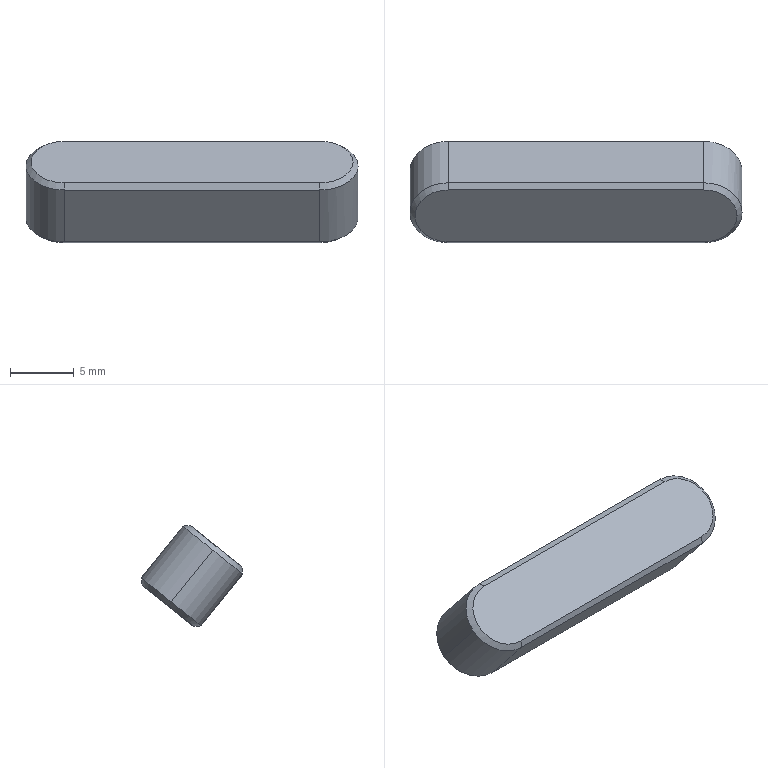Component | SolidWorks | Key6-6-32-1 | 1 solid | 17 faces | box 26 x 7.93 x 7.93 mm | volume 880 mm3 | plane 8 | cone 6 | cylinder 3 | commonest cylinder face diameters 6 x3
build123d program:
from build123d import *

# Parameters (mm, degrees)
BOSS_EXTRUDE1_DEPTH = 6
CHAMFER1_SIZE2      = 0.4
CHAMFER1_SIZE       = 0.4


with BuildPart() as part:
    # Sketch1 → Boss-Extrude1 (new body)
    with BuildSketch(Plane(origin=(0, 0, 4), x_dir=(1, 0, 0), z_dir=(0, -1, 0))):
        with BuildLine():
            Line((-3, 16), (-3, -4))
            ThreePointArc((-3, -4), (0, -7), (3, -4))
            Line((3, -4), (3, 16))
            ThreePointArc((3, 16), (0, 19), (-3, 16))
        make_face()
    extrude(amount=-BOSS_EXTRUDE1_DEPTH)

    # Chamfer1
    chamfer1_edges = [part.edges().sort_by_distance(p)[0] for p in [
        (0, 6, -3),
        (3, 6, 10),
        (0, 6, 23),
        (3, 0, 10),
        (0, 0, -3),
        (-3, 0, 10),
        (0, 0, 23),
        (-3, 6, 10),
    ]]
    chamfer(chamfer1_edges, length=CHAMFER1_SIZE, length2=CHAMFER1_SIZE2)


solid = part.part

# Placed as in the assembly
solid = solid.moved(Location((-300.42, 4.252, -5.306), (-51.293, -90, 0)))
STEP:
#1=COLOUR_RGB('',0.7922,0.8196,0.9333);
#2=FILL_AREA_STYLE_COLOUR('',#1);
#3=FILL_AREA_STYLE('',(#2));
#4=SURFACE_STYLE_FILL_AREA(#3);
#5=SURFACE_SIDE_STYLE('',(#4));
#6=SURFACE_STYLE_USAGE(.BOTH.,#5);
#7=PRESENTATION_STYLE_ASSIGNMENT((#6));
#8=CARTESIAN_POINT('',(-12.717,0.3151,-0.3932));
#9=VERTEX_POINT('',#8);
#10=CARTESIAN_POINT('',(-12.615,0.395,-0.3292));
#11=VERTEX_POINT('',#10);
#12=CARTESIAN_POINT('',(-12.615,0.3151,-0.3932));
#13=DIRECTION('',(-0.,0.6253,-0.7803));
#14=DIRECTION('',(-1.,0.,0.));
#15=AXIS2_PLACEMENT_3D('',#12,#13,#14);
#16=CIRCLE('',#15,0.1024);
#17=EDGE_CURVE('',#9,#11,#16,.T.);
#18=ORIENTED_EDGE('',*,*,#17,.F.);
#19=CARTESIAN_POINT('',(-12.733,0.3053,-0.381));
#20=VERTEX_POINT('',#19);
#21=CARTESIAN_POINT('',(-12.733,0.3053,-0.381));
#22=DIRECTION('',(-0.7071,-0.4422,0.5518));
#23=VECTOR('',#22,39.37);
#24=LINE('',#21,#23);
#25=EDGE_CURVE('',#9,#20,#24,.T.);
#26=ORIENTED_EDGE('',*,*,#25,.T.);
#27=CARTESIAN_POINT('',(-12.615,0.3975,-0.3071));
#28=VERTEX_POINT('',#27);
#29=CARTESIAN_POINT('',(-12.615,0.3053,-0.381));
#30=DIRECTION('',(0.,-0.6253,0.7803));
#31=DIRECTION('',(-1.,-0.,0.));
#32=AXIS2_PLACEMENT_3D('',#29,#30,#31);
#33=CIRCLE('',#32,0.1181);
#34=EDGE_CURVE('',#28,#20,#33,.T.);
#35=ORIENTED_EDGE('',*,*,#34,.F.);
#36=CARTESIAN_POINT('',(-12.615,0.395,-0.3292));
#37=DIRECTION('',(0.,0.1096,0.994));
#38=VECTOR('',#37,39.37);
#39=LINE('',#36,#38);
#40=EDGE_CURVE('',#11,#28,#39,.T.);
#41=ORIENTED_EDGE('',*,*,#40,.F.);
#42=EDGE_LOOP('',(#18,#26,#35,#41));
#43=FACE_OUTER_BOUND('',#42,.T.);
#44=CARTESIAN_POINT('',(-12.615,0.3053,-0.381));
#45=DIRECTION('',(0.,-0.6253,0.7803));
#46=DIRECTION('',(-1.,-0.,0.));
#47=AXIS2_PLACEMENT_3D('',#44,#45,#46);
#48=CONICAL_SURFACE('',#47,0.1181,0.7854);
#49=ADVANCED_FACE('',(#43),#48,.T.);
#50=CARTESIAN_POINT('',(-11.725,0.1674,-0.2089));
#51=VERTEX_POINT('',#50);
#52=CARTESIAN_POINT('',(-11.828,0.2473,-0.1449));
#53=VERTEX_POINT('',#52);
#54=CARTESIAN_POINT('',(-11.828,0.1674,-0.2089));
#55=DIRECTION('',(0.,-0.6253,0.7803));
#56=DIRECTION('',(-1.,-0.,0.));
#57=AXIS2_PLACEMENT_3D('',#54,#55,#56);
#58=CIRCLE('',#57,0.1024);
#59=EDGE_CURVE('',#51,#53,#58,.T.);
#60=ORIENTED_EDGE('',*,*,#59,.F.);
#61=CARTESIAN_POINT('',(-11.709,0.1773,-0.2212));
#62=VERTEX_POINT('',#61);
#63=CARTESIAN_POINT('',(-11.725,0.1674,-0.2089));
#64=DIRECTION('',(0.7071,0.4422,-0.5518));
#65=VECTOR('',#64,39.37);
#66=LINE('',#63,#65);
#67=EDGE_CURVE('',#51,#62,#66,.T.);
#68=ORIENTED_EDGE('',*,*,#67,.T.);
#69=CARTESIAN_POINT('',(-11.828,0.2694,-0.1473));
#70=VERTEX_POINT('',#69);
#71=CARTESIAN_POINT('',(-11.828,0.1773,-0.2212));
#72=DIRECTION('',(-0.,0.6253,-0.7803));
#73=DIRECTION('',(-1.,-0.,0.));
#74=AXIS2_PLACEMENT_3D('',#71,#72,#73);
#75=CIRCLE('',#74,0.1181);
#76=EDGE_CURVE('',#70,#62,#75,.T.);
#77=ORIENTED_EDGE('',*,*,#76,.F.);
#78=CARTESIAN_POINT('',(-11.828,0.2694,-0.1473));
#79=DIRECTION('',(0.,-0.994,0.1096));
#80=VECTOR('',#79,39.37);
#81=LINE('',#78,#80);
#82=EDGE_CURVE('',#70,#53,#81,.T.);
#83=ORIENTED_EDGE('',*,*,#82,.T.);
#84=EDGE_LOOP('',(#60,#68,#77,#83));
#85=FACE_OUTER_BOUND('',#84,.T.);
#86=CARTESIAN_POINT('',(-11.828,0.1674,-0.2089));
#87=DIRECTION('',(-0.,0.6253,-0.7803));
#88=DIRECTION('',(1.,0.,0.));
#89=AXIS2_PLACEMENT_3D('',#86,#87,#88);
#90=CONICAL_SURFACE('',#89,0.1024,0.7854);
#91=ADVANCED_FACE('',(#85),#90,.T.);
#92=ORIENTED_EDGE('',*,*,#34,.T.);
#93=CARTESIAN_POINT('',(-12.733,0.1773,-0.2212));
#94=VERTEX_POINT('',#93);
#95=CARTESIAN_POINT('',(-12.733,0.3151,-0.3932));
#96=DIRECTION('',(0.,-0.6253,0.7803));
#97=VECTOR('',#96,39.37);
#98=LINE('',#95,#97);
#99=EDGE_CURVE('',#20,#94,#98,.T.);
#100=ORIENTED_EDGE('',*,*,#99,.T.);
#101=CARTESIAN_POINT('',(-12.615,0.2694,-0.1473));
#102=VERTEX_POINT('',#101);
#103=CARTESIAN_POINT('',(-12.615,0.1773,-0.2212));
#104=DIRECTION('',(-0.,0.6253,-0.7803));
#105=DIRECTION('',(-1.,-0.,0.));
#106=AXIS2_PLACEMENT_3D('',#103,#104,#105);
#107=CIRCLE('',#106,0.1181);
#108=EDGE_CURVE('',#94,#102,#107,.T.);
#109=ORIENTED_EDGE('',*,*,#108,.T.);
#110=CARTESIAN_POINT('',(-12.615,0.4073,-0.3194));
#111=DIRECTION('',(0.,-0.6253,0.7803));
#112=VECTOR('',#111,39.37);
#113=LINE('',#110,#112);
#114=EDGE_CURVE('',#28,#102,#113,.T.);
#115=ORIENTED_EDGE('',*,*,#114,.F.);
#116=EDGE_LOOP('',(#92,#100,#109,#115));
#117=FACE_OUTER_BOUND('',#116,.T.);
#118=CARTESIAN_POINT('',(-12.615,0.3151,-0.3932));
#119=DIRECTION('',(0.,-0.6253,0.7803));
#120=DIRECTION('',(-1.,0.,0.));
#121=AXIS2_PLACEMENT_3D('',#118,#119,#120);
#122=CYLINDRICAL_SURFACE('',#121,0.1181);
#123=ADVANCED_FACE('',(#117),#122,.T.);
#124=CARTESIAN_POINT('',(-11.828,0.3975,-0.3071));
#125=VERTEX_POINT('',#124);
#126=CARTESIAN_POINT('',(-11.828,0.4073,-0.3194));
#127=DIRECTION('',(0.,-0.6253,0.7803));
#128=VECTOR('',#127,39.37);
#129=LINE('',#126,#128);
#130=EDGE_CURVE('',#125,#70,#129,.T.);
#131=ORIENTED_EDGE('',*,*,#130,.T.);
#132=ORIENTED_EDGE('',*,*,#76,.T.);
#133=CARTESIAN_POINT('',(-11.828,0.0851,-0.2951));
#134=VERTEX_POINT('',#133);
#135=CARTESIAN_POINT('',(-11.828,0.1773,-0.2212));
#136=DIRECTION('',(-0.,0.6253,-0.7803));
#137=DIRECTION('',(-1.,-0.,0.));
#138=AXIS2_PLACEMENT_3D('',#135,#136,#137);
#139=CIRCLE('',#138,0.1181);
#140=EDGE_CURVE('',#62,#134,#139,.T.);
#141=ORIENTED_EDGE('',*,*,#140,.T.);
#142=CARTESIAN_POINT('',(-11.828,0.2131,-0.4548));
#143=VERTEX_POINT('',#142);
#144=CARTESIAN_POINT('',(-11.828,0.223,-0.4671));
#145=DIRECTION('',(0.,-0.6253,0.7803));
#146=VECTOR('',#145,39.37);
#147=LINE('',#144,#146);
#148=EDGE_CURVE('',#143,#134,#147,.T.);
#149=ORIENTED_EDGE('',*,*,#148,.F.);
#150=CARTESIAN_POINT('',(-11.828,0.3053,-0.381));
#151=DIRECTION('',(0.,-0.6253,0.7803));
#152=DIRECTION('',(-1.,-0.,0.));
#153=AXIS2_PLACEMENT_3D('',#150,#151,#152);
#154=CIRCLE('',#153,0.1181);
#155=EDGE_CURVE('',#143,#125,#154,.T.);
#156=ORIENTED_EDGE('',*,*,#155,.T.);
#157=EDGE_LOOP('',(#131,#132,#141,#149,#156));
#158=FACE_OUTER_BOUND('',#157,.T.);
#159=CARTESIAN_POINT('',(-11.828,0.3151,-0.3932));
#160=DIRECTION('',(0.,-0.6253,0.7803));
#161=DIRECTION('',(-1.,0.,0.));
#162=AXIS2_PLACEMENT_3D('',#159,#160,#161);
#163=CYLINDRICAL_SURFACE('',#162,0.1181);
#164=ADVANCED_FACE('',(#158),#163,.T.);
#165=ORIENTED_EDGE('',*,*,#148,.T.);
#166=CARTESIAN_POINT('',(-12.615,0.0851,-0.2951));
#167=VERTEX_POINT('',#166);
#168=CARTESIAN_POINT('',(-12.615,0.0851,-0.2951));
#169=DIRECTION('',(-1.,0.,0.));
#170=VECTOR('',#169,39.37);
#171=LINE('',#168,#170);
#172=EDGE_CURVE('',#134,#167,#171,.T.);
#173=ORIENTED_EDGE('',*,*,#172,.T.);
#174=CARTESIAN_POINT('',(-12.615,0.2131,-0.4548));
#175=VERTEX_POINT('',#174);
#176=CARTESIAN_POINT('',(-12.615,0.223,-0.4671));
#177=DIRECTION('',(0.,-0.6253,0.7803));
#178=VECTOR('',#177,39.37);
#179=LINE('',#176,#178);
#180=EDGE_CURVE('',#175,#167,#179,.T.);
#181=ORIENTED_EDGE('',*,*,#180,.F.);
#182=CARTESIAN_POINT('',(-11.828,0.2131,-0.4548));
#183=DIRECTION('',(1.,-0.,-0.));
#184=VECTOR('',#183,39.37);
#185=LINE('',#182,#184);
#186=EDGE_CURVE('',#175,#143,#185,.T.);
#187=ORIENTED_EDGE('',*,*,#186,.T.);
#188=EDGE_LOOP('',(#165,#173,#181,#187));
#189=FACE_OUTER_BOUND('',#188,.T.);
#190=CARTESIAN_POINT('',(-12.615,0.223,-0.4671));
#191=DIRECTION('',(-0.,-0.7803,-0.6253));
#192=DIRECTION('',(-1.,0.,0.));
#193=AXIS2_PLACEMENT_3D('',#190,#191,#192);
#194=PLANE('',#193);
#195=ADVANCED_FACE('',(#189),#194,.T.);
#196=ORIENTED_EDGE('',*,*,#99,.F.);
#197=CARTESIAN_POINT('',(-12.615,0.3053,-0.381));
#198=DIRECTION('',(0.,-0.6253,0.7803));
#199=DIRECTION('',(-1.,-0.,0.));
#200=AXIS2_PLACEMENT_3D('',#197,#198,#199);
#201=CIRCLE('',#200,0.1181);
#202=EDGE_CURVE('',#20,#175,#201,.T.);
#203=ORIENTED_EDGE('',*,*,#202,.T.);
#204=ORIENTED_EDGE('',*,*,#180,.T.);
#205=CARTESIAN_POINT('',(-12.615,0.1773,-0.2212));
#206=DIRECTION('',(-0.,0.6253,-0.7803));
#207=DIRECTION('',(-1.,0.,0.));
#208=AXIS2_PLACEMENT_3D('',#205,#206,#207);
#209=CIRCLE('',#208,0.1181);
#210=EDGE_CURVE('',#167,#94,#209,.T.);
#211=ORIENTED_EDGE('',*,*,#210,.T.);
#212=EDGE_LOOP('',(#196,#203,#204,#211));
#213=FACE_OUTER_BOUND('',#212,.T.);
#214=CARTESIAN_POINT('',(-12.615,0.3151,-0.3932));
#215=DIRECTION('',(0.,-0.6253,0.7803));
#216=DIRECTION('',(-1.,0.,0.));
#217=AXIS2_PLACEMENT_3D('',#214,#215,#216);
#218=CYLINDRICAL_SURFACE('',#217,0.1181);
#219=ADVANCED_FACE('',(#213),#218,.T.);
#220=ORIENTED_EDGE('',*,*,#114,.T.);
#221=CARTESIAN_POINT('',(-11.828,0.2694,-0.1473));
#222=DIRECTION('',(1.,-0.,-0.));
#223=VECTOR('',#222,39.37);
#224=LINE('',#221,#223);
#225=EDGE_CURVE('',#102,#70,#224,.T.);
#226=ORIENTED_EDGE('',*,*,#225,.T.);
#227=ORIENTED_EDGE('',*,*,#130,.F.);
#228=CARTESIAN_POINT('',(-12.615,0.3975,-0.3071));
#229=DIRECTION('',(-1.,0.,0.));
#230=VECTOR('',#229,39.37);
#231=LINE('',#228,#230);
#232=EDGE_CURVE('',#125,#28,#231,.T.);
#233=ORIENTED_EDGE('',*,*,#232,.T.);
#234=EDGE_LOOP('',(#220,#226,#227,#233));
#235=FACE_OUTER_BOUND('',#234,.T.);
#236=CARTESIAN_POINT('',(-11.828,0.4073,-0.3194));
#237=DIRECTION('',(0.,0.7803,0.6253));
#238=DIRECTION('',(1.,-0.,-0.));
#239=AXIS2_PLACEMENT_3D('',#236,#237,#238);
#240=PLANE('',#239);
#241=ADVANCED_FACE('',(#235),#240,.T.);
#242=CARTESIAN_POINT('',(-12.615,0.2353,-0.4573));
#243=VERTEX_POINT('',#242);
#244=CARTESIAN_POINT('',(-12.615,0.3151,-0.3932));
#245=DIRECTION('',(-0.,0.6253,-0.7803));
#246=DIRECTION('',(-1.,0.,0.));
#247=AXIS2_PLACEMENT_3D('',#244,#245,#246);
#248=CIRCLE('',#247,0.1024);
#249=EDGE_CURVE('',#243,#9,#248,.T.);
#250=ORIENTED_EDGE('',*,*,#249,.T.);
#251=ORIENTED_EDGE('',*,*,#17,.T.);
#252=CARTESIAN_POINT('',(-11.828,0.395,-0.3292));
#253=VERTEX_POINT('',#252);
#254=CARTESIAN_POINT('',(-11.828,0.395,-0.3292));
#255=DIRECTION('',(1.,-0.,-0.));
#256=VECTOR('',#255,39.37);
#257=LINE('',#254,#256);
#258=EDGE_CURVE('',#11,#253,#257,.T.);
#259=ORIENTED_EDGE('',*,*,#258,.T.);
#260=CARTESIAN_POINT('',(-11.828,0.2353,-0.4573));
#261=VERTEX_POINT('',#260);
#262=CARTESIAN_POINT('',(-11.828,0.3151,-0.3932));
#263=DIRECTION('',(-0.,0.6253,-0.7803));
#264=DIRECTION('',(-1.,0.,0.));
#265=AXIS2_PLACEMENT_3D('',#262,#263,#264);
#266=CIRCLE('',#265,0.1024);
#267=EDGE_CURVE('',#253,#261,#266,.T.);
#268=ORIENTED_EDGE('',*,*,#267,.T.);
#269=CARTESIAN_POINT('',(-12.615,0.2353,-0.4573));
#270=DIRECTION('',(-1.,0.,0.));
#271=VECTOR('',#270,39.37);
#272=LINE('',#269,#271);
#273=EDGE_CURVE('',#261,#243,#272,.T.);
#274=ORIENTED_EDGE('',*,*,#273,.T.);
#275=EDGE_LOOP('',(#250,#251,#259,#268,#274));
#276=FACE_OUTER_BOUND('',#275,.T.);
#277=CARTESIAN_POINT('',(-11.828,0.3151,-0.3932));
#278=DIRECTION('',(-0.,-0.6253,0.7803));
#279=DIRECTION('',(-1.,-0.,-0.));
#280=AXIS2_PLACEMENT_3D('',#277,#278,#279);
#281=PLANE('',#280);
#282=ADVANCED_FACE('',(#276),#281,.F.);
#283=CARTESIAN_POINT('',(-12.615,0.2473,-0.1449));
#284=VERTEX_POINT('',#283);
#285=CARTESIAN_POINT('',(-12.615,0.08754,-0.2729));
#286=VERTEX_POINT('',#285);
#287=CARTESIAN_POINT('',(-12.615,0.1674,-0.2089));
#288=DIRECTION('',(0.,-0.6253,0.7803));
#289=DIRECTION('',(-1.,-0.,0.));
#290=AXIS2_PLACEMENT_3D('',#287,#288,#289);
#291=CIRCLE('',#290,0.1024);
#292=EDGE_CURVE('',#284,#286,#291,.T.);
#293=ORIENTED_EDGE('',*,*,#292,.T.);
#294=CARTESIAN_POINT('',(-11.828,0.08754,-0.2729));
#295=VERTEX_POINT('',#294);
#296=CARTESIAN_POINT('',(-11.828,0.08754,-0.2729));
#297=DIRECTION('',(1.,-0.,-0.));
#298=VECTOR('',#297,39.37);
#299=LINE('',#296,#298);
#300=EDGE_CURVE('',#286,#295,#299,.T.);
#301=ORIENTED_EDGE('',*,*,#300,.T.);
#302=CARTESIAN_POINT('',(-11.828,0.1674,-0.2089));
#303=DIRECTION('',(0.,-0.6253,0.7803));
#304=DIRECTION('',(-1.,-0.,0.));
#305=AXIS2_PLACEMENT_3D('',#302,#303,#304);
#306=CIRCLE('',#305,0.1024);
#307=EDGE_CURVE('',#295,#51,#306,.T.);
#308=ORIENTED_EDGE('',*,*,#307,.T.);
#309=ORIENTED_EDGE('',*,*,#59,.T.);
#310=CARTESIAN_POINT('',(-11.828,0.2473,-0.1449));
#311=DIRECTION('',(-1.,0.,0.));
#312=VECTOR('',#311,39.37);
#313=LINE('',#310,#312);
#314=EDGE_CURVE('',#53,#284,#313,.T.);
#315=ORIENTED_EDGE('',*,*,#314,.T.);
#316=EDGE_LOOP('',(#293,#301,#308,#309,#315));
#317=FACE_OUTER_BOUND('',#316,.T.);
#318=CARTESIAN_POINT('',(-11.828,0.1674,-0.2089));
#319=DIRECTION('',(-0.,-0.6253,0.7803));
#320=DIRECTION('',(-1.,-0.,-0.));
#321=AXIS2_PLACEMENT_3D('',#318,#319,#320);
#322=PLANE('',#321);
#323=ADVANCED_FACE('',(#317),#322,.T.);
#324=ORIENTED_EDGE('',*,*,#82,.F.);
#325=ORIENTED_EDGE('',*,*,#225,.F.);
#326=CARTESIAN_POINT('',(-12.615,0.2473,-0.1449));
#327=DIRECTION('',(-0.,0.994,-0.1096));
#328=VECTOR('',#327,39.37);
#329=LINE('',#326,#328);
#330=EDGE_CURVE('',#284,#102,#329,.T.);
#331=ORIENTED_EDGE('',*,*,#330,.F.);
#332=ORIENTED_EDGE('',*,*,#314,.F.);
#333=EDGE_LOOP('',(#324,#325,#331,#332));
#334=FACE_OUTER_BOUND('',#333,.T.);
#335=CARTESIAN_POINT('',(-11.828,0.2473,-0.1449));
#336=DIRECTION('',(-0.,-0.1096,-0.994));
#337=DIRECTION('',(-1.,0.,0.));
#338=AXIS2_PLACEMENT_3D('',#335,#336,#337);
#339=PLANE('',#338);
#340=ADVANCED_FACE('',(#334),#339,.F.);
#341=ORIENTED_EDGE('',*,*,#330,.T.);
#342=ORIENTED_EDGE('',*,*,#108,.F.);
#343=ORIENTED_EDGE('',*,*,#210,.F.);
#344=CARTESIAN_POINT('',(-12.615,0.08754,-0.2729));
#345=DIRECTION('',(-0.,-0.1096,-0.994));
#346=VECTOR('',#345,39.37);
#347=LINE('',#344,#346);
#348=EDGE_CURVE('',#286,#167,#347,.T.);
#349=ORIENTED_EDGE('',*,*,#348,.F.);
#350=ORIENTED_EDGE('',*,*,#292,.F.);
#351=EDGE_LOOP('',(#341,#342,#343,#349,#350));
#352=FACE_OUTER_BOUND('',#351,.T.);
#353=CARTESIAN_POINT('',(-12.615,0.1674,-0.2089));
#354=DIRECTION('',(-0.,0.6253,-0.7803));
#355=DIRECTION('',(1.,0.,0.));
#356=AXIS2_PLACEMENT_3D('',#353,#354,#355);
#357=CONICAL_SURFACE('',#356,0.1024,0.7854);
#358=ADVANCED_FACE('',(#352),#357,.T.);
#359=ORIENTED_EDGE('',*,*,#67,.F.);
#360=ORIENTED_EDGE('',*,*,#307,.F.);
#361=CARTESIAN_POINT('',(-11.828,0.0851,-0.2951));
#362=DIRECTION('',(-0.,0.1096,0.994));
#363=VECTOR('',#362,39.37);
#364=LINE('',#361,#363);
#365=EDGE_CURVE('',#134,#295,#364,.T.);
#366=ORIENTED_EDGE('',*,*,#365,.F.);
#367=ORIENTED_EDGE('',*,*,#140,.F.);
#368=EDGE_LOOP('',(#359,#360,#366,#367));
#369=FACE_OUTER_BOUND('',#368,.T.);
#370=CARTESIAN_POINT('',(-11.828,0.1674,-0.2089));
#371=DIRECTION('',(-0.,0.6253,-0.7803));
#372=DIRECTION('',(1.,0.,0.));
#373=AXIS2_PLACEMENT_3D('',#370,#371,#372);
#374=CONICAL_SURFACE('',#373,0.1024,0.7854);
#375=ADVANCED_FACE('',(#369),#374,.T.);
#376=ORIENTED_EDGE('',*,*,#348,.T.);
#377=ORIENTED_EDGE('',*,*,#172,.F.);
#378=ORIENTED_EDGE('',*,*,#365,.T.);
#379=ORIENTED_EDGE('',*,*,#300,.F.);
#380=EDGE_LOOP('',(#376,#377,#378,#379));
#381=FACE_OUTER_BOUND('',#380,.T.);
#382=CARTESIAN_POINT('',(-11.828,0.08754,-0.2729));
#383=DIRECTION('',(0.,0.994,-0.1096));
#384=DIRECTION('',(1.,-0.,-0.));
#385=AXIS2_PLACEMENT_3D('',#382,#383,#384);
#386=PLANE('',#385);
#387=ADVANCED_FACE('',(#381),#386,.F.);
#388=CARTESIAN_POINT('',(-12.615,0.2353,-0.4573));
#389=DIRECTION('',(0.,-0.994,0.1096));
#390=VECTOR('',#389,39.37);
#391=LINE('',#388,#390);
#392=EDGE_CURVE('',#243,#175,#391,.T.);
#393=ORIENTED_EDGE('',*,*,#392,.F.);
#394=ORIENTED_EDGE('',*,*,#273,.F.);
#395=CARTESIAN_POINT('',(-11.828,0.2131,-0.4548));
#396=DIRECTION('',(-0.,0.994,-0.1096));
#397=VECTOR('',#396,39.37);
#398=LINE('',#395,#397);
#399=EDGE_CURVE('',#143,#261,#398,.T.);
#400=ORIENTED_EDGE('',*,*,#399,.F.);
#401=ORIENTED_EDGE('',*,*,#186,.F.);
#402=EDGE_LOOP('',(#393,#394,#400,#401));
#403=FACE_OUTER_BOUND('',#402,.T.);
#404=CARTESIAN_POINT('',(-12.615,0.2131,-0.4548));
#405=DIRECTION('',(-0.,-0.1096,-0.994));
#406=DIRECTION('',(-1.,0.,0.));
#407=AXIS2_PLACEMENT_3D('',#404,#405,#406);
#408=PLANE('',#407);
#409=ADVANCED_FACE('',(#403),#408,.T.);
#410=ORIENTED_EDGE('',*,*,#399,.T.);
#411=ORIENTED_EDGE('',*,*,#267,.F.);
#412=CARTESIAN_POINT('',(-11.828,0.3975,-0.3071));
#413=DIRECTION('',(0.,-0.1096,-0.994));
#414=VECTOR('',#413,39.37);
#415=LINE('',#412,#414);
#416=EDGE_CURVE('',#125,#253,#415,.T.);
#417=ORIENTED_EDGE('',*,*,#416,.F.);
#418=ORIENTED_EDGE('',*,*,#155,.F.);
#419=EDGE_LOOP('',(#410,#411,#417,#418));
#420=FACE_OUTER_BOUND('',#419,.T.);
#421=CARTESIAN_POINT('',(-11.828,0.3053,-0.381));
#422=DIRECTION('',(0.,-0.6253,0.7803));
#423=DIRECTION('',(-1.,-0.,0.));
#424=AXIS2_PLACEMENT_3D('',#421,#422,#423);
#425=CONICAL_SURFACE('',#424,0.1181,0.7854);
#426=ADVANCED_FACE('',(#420),#425,.T.);
#427=ORIENTED_EDGE('',*,*,#25,.F.);
#428=ORIENTED_EDGE('',*,*,#249,.F.);
#429=ORIENTED_EDGE('',*,*,#392,.T.);
#430=ORIENTED_EDGE('',*,*,#202,.F.);
#431=EDGE_LOOP('',(#427,#428,#429,#430));
#432=FACE_OUTER_BOUND('',#431,.T.);
#433=CARTESIAN_POINT('',(-12.615,0.3053,-0.381));
#434=DIRECTION('',(0.,-0.6253,0.7803));
#435=DIRECTION('',(-1.,-0.,0.));
#436=AXIS2_PLACEMENT_3D('',#433,#434,#435);
#437=CONICAL_SURFACE('',#436,0.1181,0.7854);
#438=ADVANCED_FACE('',(#432),#437,.T.);
#439=ORIENTED_EDGE('',*,*,#416,.T.);
#440=ORIENTED_EDGE('',*,*,#258,.F.);
#441=ORIENTED_EDGE('',*,*,#40,.T.);
#442=ORIENTED_EDGE('',*,*,#232,.F.);
#443=EDGE_LOOP('',(#439,#440,#441,#442));
#444=FACE_OUTER_BOUND('',#443,.T.);
#445=CARTESIAN_POINT('',(-11.828,0.3975,-0.3071));
#446=DIRECTION('',(0.,0.994,-0.1096));
#447=DIRECTION('',(1.,-0.,-0.));
#448=AXIS2_PLACEMENT_3D('',#445,#446,#447);
#449=PLANE('',#448);
#450=ADVANCED_FACE('',(#444),#449,.T.);
#451=CLOSED_SHELL('',(#49,#91,#123,#164,#195,#219,#241,#282,#323,#340,#358,#375,#387,#409,#426,#438,#450));
#452=MANIFOLD_SOLID_BREP('',#451);
#453=STYLED_ITEM('',(#7),#452);
#454=PRESENTATION_LAYER_ASSIGNMENT('','',(#453));
#455=CARTESIAN_POINT('',(0.,0.,0.));
#456=DIRECTION('',(0.,0.,1.));
#457=DIRECTION('',(1.,0.,0.));
#458=AXIS2_PLACEMENT_3D('',#455,#456,#457);
#459=(LENGTH_UNIT()NAMED_UNIT(*)SI_UNIT($,.METRE.));
#460=LENGTH_MEASURE_WITH_UNIT(LENGTH_MEASURE(0.0254),#459);
#461=DIMENSIONAL_EXPONENTS(1.,0.,0.,0.,0.,0.,0.);
#462=(CONVERSION_BASED_UNIT('',#460)LENGTH_UNIT()NAMED_UNIT(#461));
#463=UNCERTAINTY_MEASURE_WITH_UNIT(LENGTH_MEASURE(0.00001),#462,'','');
#464=(NAMED_UNIT(*)PLANE_ANGLE_UNIT()SI_UNIT($,.RADIAN.));
#465=(NAMED_UNIT(*)SI_UNIT($,.STERADIAN.)SOLID_ANGLE_UNIT());
#466=(GEOMETRIC_REPRESENTATION_CONTEXT(3)GLOBAL_UNCERTAINTY_ASSIGNED_CONTEXT((#463))GLOBAL_UNIT_ASSIGNED_CONTEXT((#462,#464,#465))REPRESENTATION_CONTEXT('',''));
#467=ADVANCED_BREP_SHAPE_REPRESENTATION('',(#452,#458),#466);
#468=(LENGTH_UNIT()NAMED_UNIT(*)SI_UNIT($,.METRE.));
#469=LENGTH_MEASURE_WITH_UNIT(LENGTH_MEASURE(0.0254),#468);
#470=DIMENSIONAL_EXPONENTS(1.,0.,0.,0.,0.,0.,0.);
#471=(CONVERSION_BASED_UNIT('',#469)LENGTH_UNIT()NAMED_UNIT(#470));
#472=UNCERTAINTY_MEASURE_WITH_UNIT(LENGTH_MEASURE(0.00001),#471,'','');
#473=(NAMED_UNIT(*)PLANE_ANGLE_UNIT()SI_UNIT($,.RADIAN.));
#474=(NAMED_UNIT(*)SI_UNIT($,.STERADIAN.)SOLID_ANGLE_UNIT());
#475=(GEOMETRIC_REPRESENTATION_CONTEXT(3)GLOBAL_UNCERTAINTY_ASSIGNED_CONTEXT((#472))GLOBAL_UNIT_ASSIGNED_CONTEXT((#471,#473,#474))REPRESENTATION_CONTEXT('',''));
#476=MECHANICAL_DESIGN_GEOMETRIC_PRESENTATION_REPRESENTATION('',(#453),#475);